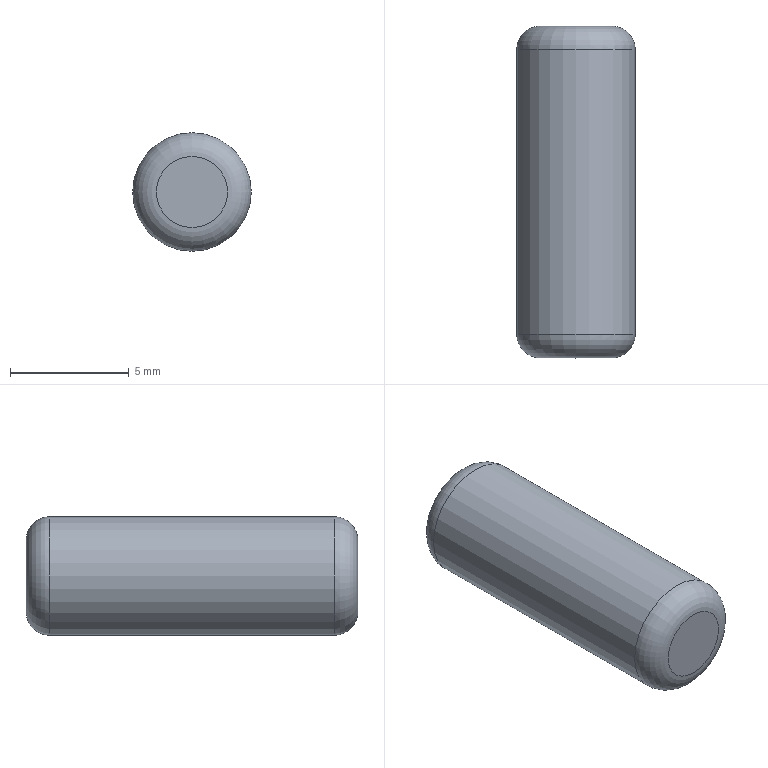Component | NX | M5_2 | 1 solid | 5 faces | box 5 x 14 x 5 mm | volume 269 mm3 | plane 2 | torus 2 | cylinder 1 | commonest cylinder face diameters 5 x1
STEP:
#1=CARTESIAN_POINT('',(0.,0.,0.));
#2=DIRECTION('',(0.,0.,1.));
#3=DIRECTION('',(1.,0.,0.));
#4=AXIS2_PLACEMENT_3D('',#1,#2,#3);
#5=CARTESIAN_POINT('',(6.,7.,205.511));
#6=VERTEX_POINT('',#5);
#7=CARTESIAN_POINT('',(6.,7.,204.011));
#8=DIRECTION('',(0.,-1.,0.));
#9=DIRECTION('',(0.,0.,1.));
#10=AXIS2_PLACEMENT_3D('',#7,#8,#9);
#11=CIRCLE('',#10,1.5);
#12=CARTESIAN_POINT('',(6.,7.,205.511));
#13=DIRECTION('',(0.,1.,0.));
#14=DIRECTION('',(0.,0.,-1.));
#15=AXIS2_PLACEMENT_3D('',#12,#13,#14);
#16=PLANE('',#15);
#17=CARTESIAN_POINT('',(0.,0.));
#18=CARTESIAN_POINT('',(0.,2.598));
#19=CARTESIAN_POINT('',(2.25,1.299));
#20=CARTESIAN_POINT('',(4.5,0.));
#21=CARTESIAN_POINT('',(2.25,-1.299));
#22=CARTESIAN_POINT('',(0.,-2.598));
#23=CARTESIAN_POINT('',(0.,0.));
#24=(BOUNDED_CURVE()B_SPLINE_CURVE(2,(#17,#18,#19,#20,#21,#22,#23),.UNSPECIFIED.,.T.,.F.)B_SPLINE_CURVE_WITH_KNOTS((1,2,2,2,2,1),(-2.094,0.,2.094,4.189,6.283,8.378),.UNSPECIFIED.)CURVE()GEOMETRIC_REPRESENTATION_ITEM()RATIONAL_B_SPLINE_CURVE((1.,0.5,1.,0.5,1.,0.5,1.))REPRESENTATION_ITEM(''));
#25=(GEOMETRIC_REPRESENTATION_CONTEXT(2)PARAMETRIC_REPRESENTATION_CONTEXT()REPRESENTATION_CONTEXT('',''));
#26=DEFINITIONAL_REPRESENTATION('',(#24),#25);
#27=PCURVE('',#16,#26);
#28=CARTESIAN_POINT('',(6.,6.,204.011));
#29=DIRECTION('',(0.,-1.,0.));
#30=DIRECTION('',(0.,0.,1.));
#31=AXIS2_PLACEMENT_3D('',#28,#29,#30);
#32=TOROIDAL_SURFACE('',#31,1.5,1.);
#33=CARTESIAN_POINT('',(0.,4.712));
#34=DIRECTION('',(1.,0.));
#35=VECTOR('',#34,1.);
#36=LINE('',#33,#35);
#37=(GEOMETRIC_REPRESENTATION_CONTEXT(2)PARAMETRIC_REPRESENTATION_CONTEXT()REPRESENTATION_CONTEXT('',''));
#38=DEFINITIONAL_REPRESENTATION('',(#36),#37);
#39=PCURVE('',#32,#38);
#40=SURFACE_CURVE('',#11,(#27,#39),.PCURVE_S1.);
#41=EDGE_CURVE('',#6,#6,#40,.T.);
#42=ORIENTED_EDGE('',*,*,#41,.F.);
#43=EDGE_LOOP('',(#42));
#44=FACE_BOUND('',#43,.T.);
#45=ADVANCED_FACE('',(#44),#16,.T.);
#46=ORIENTED_EDGE('',*,*,#41,.T.);
#47=CARTESIAN_POINT('',(6.,6.,206.511));
#48=VERTEX_POINT('',#47);
#49=CARTESIAN_POINT('',(6.,7.,205.511));
#50=CARTESIAN_POINT('',(6.,7.,205.779));
#51=CARTESIAN_POINT('',(6.,6.915,206.039));
#52=CARTESIAN_POINT('',(6.,6.752,206.263));
#53=CARTESIAN_POINT('',(6.,6.528,206.426));
#54=CARTESIAN_POINT('',(6.,6.267,206.511));
#55=CARTESIAN_POINT('',(6.,6.,206.511));
#56=(BOUNDED_CURVE()B_SPLINE_CURVE(6,(#49,#50,#51,#52,#53,#54,#55),.UNSPECIFIED.,.F.,.F.)B_SPLINE_CURVE_WITH_KNOTS((7,7),(4.712,6.283),.PIECEWISE_BEZIER_KNOTS.)CURVE()GEOMETRIC_REPRESENTATION_ITEM()RATIONAL_B_SPLINE_CURVE((1.031,1.01,0.9979,0.994,0.9979,1.01,1.031))REPRESENTATION_ITEM(''));
#57=CARTESIAN_POINT('',(6.283,0.));
#58=DIRECTION('',(0.,1.));
#59=VECTOR('',#58,1.);
#60=LINE('',#57,#59);
#61=(GEOMETRIC_REPRESENTATION_CONTEXT(2)PARAMETRIC_REPRESENTATION_CONTEXT()REPRESENTATION_CONTEXT('',''));
#62=DEFINITIONAL_REPRESENTATION('',(#60),#61);
#63=PCURVE('',#32,#62);
#64=CARTESIAN_POINT('',(0.,0.));
#65=DIRECTION('',(0.,1.));
#66=VECTOR('',#65,1.);
#67=LINE('',#64,#66);
#68=(GEOMETRIC_REPRESENTATION_CONTEXT(2)PARAMETRIC_REPRESENTATION_CONTEXT()REPRESENTATION_CONTEXT('',''));
#69=DEFINITIONAL_REPRESENTATION('',(#67),#68);
#70=PCURVE('',#32,#69);
#71=SEAM_CURVE('',#56,(#63,#70),.PCURVE_S1.);
#72=EDGE_CURVE('',#6,#48,#71,.T.);
#73=ORIENTED_EDGE('',*,*,#72,.T.);
#74=CARTESIAN_POINT('',(6.,6.,204.011));
#75=DIRECTION('',(0.,-1.,0.));
#76=DIRECTION('',(0.,0.,1.));
#77=AXIS2_PLACEMENT_3D('',#74,#75,#76);
#78=CIRCLE('',#77,2.5);
#79=CARTESIAN_POINT('',(0.,6.283));
#80=DIRECTION('',(1.,0.));
#81=VECTOR('',#80,1.);
#82=LINE('',#79,#81);
#83=(GEOMETRIC_REPRESENTATION_CONTEXT(2)PARAMETRIC_REPRESENTATION_CONTEXT()REPRESENTATION_CONTEXT('',''));
#84=DEFINITIONAL_REPRESENTATION('',(#82),#83);
#85=PCURVE('',#32,#84);
#86=CARTESIAN_POINT('',(6.,-23.,204.011));
#87=DIRECTION('',(0.,-1.,0.));
#88=DIRECTION('',(0.,0.,1.));
#89=AXIS2_PLACEMENT_3D('',#86,#87,#88);
#90=CYLINDRICAL_SURFACE('',#89,2.5);
#91=CARTESIAN_POINT('',(0.,-29.));
#92=DIRECTION('',(1.,0.));
#93=VECTOR('',#92,1.);
#94=LINE('',#91,#93);
#95=(GEOMETRIC_REPRESENTATION_CONTEXT(2)PARAMETRIC_REPRESENTATION_CONTEXT()REPRESENTATION_CONTEXT('',''));
#96=DEFINITIONAL_REPRESENTATION('',(#94),#95);
#97=PCURVE('',#90,#96);
#98=SURFACE_CURVE('',#78,(#85,#97),.PCURVE_S1.);
#99=EDGE_CURVE('',#48,#48,#98,.T.);
#100=ORIENTED_EDGE('',*,*,#99,.F.);
#101=ORIENTED_EDGE('',*,*,#72,.F.);
#102=EDGE_LOOP('',(#46,#73,#100,#101));
#103=FACE_BOUND('',#102,.T.);
#104=ADVANCED_FACE('',(#103),#32,.T.);
#105=ORIENTED_EDGE('',*,*,#99,.T.);
#106=CARTESIAN_POINT('',(6.,-6.,206.511));
#107=VERTEX_POINT('',#106);
#108=CARTESIAN_POINT('',(6.,6.,206.511));
#109=CARTESIAN_POINT('',(6.,-6.,206.511));
#110=B_SPLINE_CURVE_WITH_KNOTS('',1,(#108,#109),.UNSPECIFIED.,.F.,.F.,(2,2),(-29.,-17.),.PIECEWISE_BEZIER_KNOTS.);
#111=CARTESIAN_POINT('',(6.283,0.));
#112=DIRECTION('',(0.,1.));
#113=VECTOR('',#112,1.);
#114=LINE('',#111,#113);
#115=(GEOMETRIC_REPRESENTATION_CONTEXT(2)PARAMETRIC_REPRESENTATION_CONTEXT()REPRESENTATION_CONTEXT('',''));
#116=DEFINITIONAL_REPRESENTATION('',(#114),#115);
#117=PCURVE('',#90,#116);
#118=CARTESIAN_POINT('',(0.,0.));
#119=DIRECTION('',(0.,1.));
#120=VECTOR('',#119,1.);
#121=LINE('',#118,#120);
#122=(GEOMETRIC_REPRESENTATION_CONTEXT(2)PARAMETRIC_REPRESENTATION_CONTEXT()REPRESENTATION_CONTEXT('',''));
#123=DEFINITIONAL_REPRESENTATION('',(#121),#122);
#124=PCURVE('',#90,#123);
#125=SEAM_CURVE('',#110,(#117,#124),.PCURVE_S1.);
#126=EDGE_CURVE('',#48,#107,#125,.T.);
#127=ORIENTED_EDGE('',*,*,#126,.T.);
#128=CARTESIAN_POINT('',(6.,-6.,204.011));
#129=DIRECTION('',(0.,-1.,0.));
#130=DIRECTION('',(0.,0.,1.));
#131=AXIS2_PLACEMENT_3D('',#128,#129,#130);
#132=CIRCLE('',#131,2.5);
#133=CARTESIAN_POINT('',(0.,-17.));
#134=DIRECTION('',(1.,0.));
#135=VECTOR('',#134,1.);
#136=LINE('',#133,#135);
#137=(GEOMETRIC_REPRESENTATION_CONTEXT(2)PARAMETRIC_REPRESENTATION_CONTEXT()REPRESENTATION_CONTEXT('',''));
#138=DEFINITIONAL_REPRESENTATION('',(#136),#137);
#139=PCURVE('',#90,#138);
#140=CARTESIAN_POINT('',(6.,-6.,204.011));
#141=DIRECTION('',(0.,-1.,0.));
#142=DIRECTION('',(0.,0.,1.));
#143=AXIS2_PLACEMENT_3D('',#140,#141,#142);
#144=TOROIDAL_SURFACE('',#143,1.5,1.);
#145=CARTESIAN_POINT('',(0.,6.283));
#146=DIRECTION('',(1.,0.));
#147=VECTOR('',#146,1.);
#148=LINE('',#145,#147);
#149=(GEOMETRIC_REPRESENTATION_CONTEXT(2)PARAMETRIC_REPRESENTATION_CONTEXT()REPRESENTATION_CONTEXT('',''));
#150=DEFINITIONAL_REPRESENTATION('',(#148),#149);
#151=PCURVE('',#144,#150);
#152=SURFACE_CURVE('',#132,(#139,#151),.PCURVE_S1.);
#153=EDGE_CURVE('',#107,#107,#152,.T.);
#154=ORIENTED_EDGE('',*,*,#153,.F.);
#155=ORIENTED_EDGE('',*,*,#126,.F.);
#156=EDGE_LOOP('',(#105,#127,#154,#155));
#157=FACE_BOUND('',#156,.T.);
#158=ADVANCED_FACE('',(#157),#90,.T.);
#159=ORIENTED_EDGE('',*,*,#153,.T.);
#160=CARTESIAN_POINT('',(6.,-7.,205.511));
#161=VERTEX_POINT('',#160);
#162=CARTESIAN_POINT('',(6.,-6.,206.511));
#163=CARTESIAN_POINT('',(6.,-6.267,206.511));
#164=CARTESIAN_POINT('',(6.,-6.528,206.426));
#165=CARTESIAN_POINT('',(6.,-6.752,206.263));
#166=CARTESIAN_POINT('',(6.,-6.915,206.039));
#167=CARTESIAN_POINT('',(6.,-7.,205.779));
#168=CARTESIAN_POINT('',(6.,-7.,205.511));
#169=(BOUNDED_CURVE()B_SPLINE_CURVE(6,(#162,#163,#164,#165,#166,#167,#168),.UNSPECIFIED.,.F.,.F.)B_SPLINE_CURVE_WITH_KNOTS((7,7),(0.,1.571),.PIECEWISE_BEZIER_KNOTS.)CURVE()GEOMETRIC_REPRESENTATION_ITEM()RATIONAL_B_SPLINE_CURVE((1.031,1.01,0.9979,0.994,0.9979,1.01,1.031))REPRESENTATION_ITEM(''));
#170=CARTESIAN_POINT('',(6.283,6.283));
#171=DIRECTION('',(0.,1.));
#172=VECTOR('',#171,1.);
#173=LINE('',#170,#172);
#174=(GEOMETRIC_REPRESENTATION_CONTEXT(2)PARAMETRIC_REPRESENTATION_CONTEXT()REPRESENTATION_CONTEXT('',''));
#175=DEFINITIONAL_REPRESENTATION('',(#173),#174);
#176=PCURVE('',#144,#175);
#177=CARTESIAN_POINT('',(0.,6.283));
#178=DIRECTION('',(0.,1.));
#179=VECTOR('',#178,1.);
#180=LINE('',#177,#179);
#181=(GEOMETRIC_REPRESENTATION_CONTEXT(2)PARAMETRIC_REPRESENTATION_CONTEXT()REPRESENTATION_CONTEXT('',''));
#182=DEFINITIONAL_REPRESENTATION('',(#180),#181);
#183=PCURVE('',#144,#182);
#184=SEAM_CURVE('',#169,(#176,#183),.PCURVE_S1.);
#185=EDGE_CURVE('',#107,#161,#184,.T.);
#186=ORIENTED_EDGE('',*,*,#185,.T.);
#187=CARTESIAN_POINT('',(6.,-7.,204.011));
#188=DIRECTION('',(0.,-1.,0.));
#189=DIRECTION('',(0.,0.,1.));
#190=AXIS2_PLACEMENT_3D('',#187,#188,#189);
#191=CIRCLE('',#190,1.5);
#192=CARTESIAN_POINT('',(0.,7.854));
#193=DIRECTION('',(1.,0.));
#194=VECTOR('',#193,1.);
#195=LINE('',#192,#194);
#196=(GEOMETRIC_REPRESENTATION_CONTEXT(2)PARAMETRIC_REPRESENTATION_CONTEXT()REPRESENTATION_CONTEXT('',''));
#197=DEFINITIONAL_REPRESENTATION('',(#195),#196);
#198=PCURVE('',#144,#197);
#199=CARTESIAN_POINT('',(6.,-7.,204.011));
#200=DIRECTION('',(0.,-1.,0.));
#201=DIRECTION('',(0.,0.,1.));
#202=AXIS2_PLACEMENT_3D('',#199,#200,#201);
#203=PLANE('',#202);
#204=CARTESIAN_POINT('',(0.,0.));
#205=DIRECTION('',(1.,0.));
#206=AXIS2_PLACEMENT_2D('',#204,#205);
#207=CIRCLE('',#206,1.5);
#208=(GEOMETRIC_REPRESENTATION_CONTEXT(2)PARAMETRIC_REPRESENTATION_CONTEXT()REPRESENTATION_CONTEXT('',''));
#209=DEFINITIONAL_REPRESENTATION('',(#207),#208);
#210=PCURVE('',#203,#209);
#211=SURFACE_CURVE('',#191,(#198,#210),.PCURVE_S1.);
#212=EDGE_CURVE('',#161,#161,#211,.T.);
#213=ORIENTED_EDGE('',*,*,#212,.F.);
#214=ORIENTED_EDGE('',*,*,#185,.F.);
#215=EDGE_LOOP('',(#159,#186,#213,#214));
#216=FACE_BOUND('',#215,.T.);
#217=ADVANCED_FACE('',(#216),#144,.T.);
#218=ORIENTED_EDGE('',*,*,#212,.T.);
#219=EDGE_LOOP('',(#218));
#220=FACE_BOUND('',#219,.T.);
#221=ADVANCED_FACE('',(#220),#203,.T.);
#222=CLOSED_SHELL('',(#45,#104,#158,#217,#221));
#223=MANIFOLD_SOLID_BREP('',#222);
#224=(LENGTH_UNIT()NAMED_UNIT(*)SI_UNIT(.MILLI.,.METRE.));
#225=UNCERTAINTY_MEASURE_WITH_UNIT(LENGTH_MEASURE(0.00001),#224,'','');
#226=(NAMED_UNIT(*)PLANE_ANGLE_UNIT()SI_UNIT($,.RADIAN.));
#227=(NAMED_UNIT(*)SI_UNIT($,.STERADIAN.)SOLID_ANGLE_UNIT());
#228=(GEOMETRIC_REPRESENTATION_CONTEXT(3)GLOBAL_UNCERTAINTY_ASSIGNED_CONTEXT((#225))GLOBAL_UNIT_ASSIGNED_CONTEXT((#224,#226,#227))REPRESENTATION_CONTEXT('',''));
#229=ADVANCED_BREP_SHAPE_REPRESENTATION('',(#4,#223),#228);